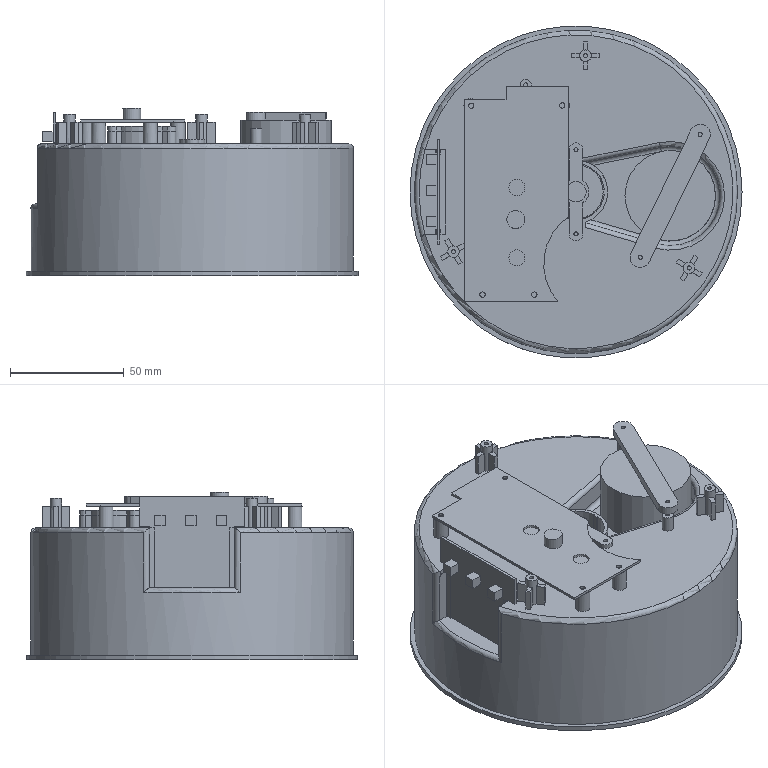Assembly | NX | mm | 9 component files | 9 solids | 350 faces | box 146 x 146 x 73.54 mm | volume 144346 mm3 | plane 205 | cylinder 113 | torus 18 | spline 7 | sphere 7 | commonest cylinder face diameters 4 x27 1.8 x17 2.35 x8 4.915 x6 24 x6 5 x5 23.94 x4 24.9 x4
Bill of materials:
unnamed part 1 | 1 |  | Thin flat plate with a T-shaped outline: a wider rectangular head band over a narrower rectangular body. The edge views show small rectangular blocks standing out from one face.
unnamed part 2 | 1 |  | Flat bar with rounded ends and a small through hole near each end. At the middle is a ring-shaped pad over a hollow cylindrical tube that sticks out from one side of the bar.
unnamed part 3 | 1 |  | Thin round disc with three rounded ears spaced about evenly around the edge. Each ear has a small through hole.
unnamed part 4 | 1 |  | Long, thin flat bar with rounded ends and a small through hole near each end.
unnamed part 5 | 1 |  | Wide, short cylindrical housing with a closed top and a narrow lip around the base. The top carries several upright features: small round posts, cross-shaped posts, a central boss with mounting lugs, and a hollow tube boss with a raised teardrop-shaped wall running from it.
unnamed part 6 | 1 |  | Solid cylinder with a short, narrower step collar on one end and a thin round shaft extending from the collar on the same axis.
unnamed part 7 | 1 |  | Plain solid cylinder, wider than it is tall.
unnamed part 8 | 1 |  | Thin flat plate, roughly rectangular, with a step-shaped notch along one short edge and a large curved (concave) cutout at one corner. It has two larger through holes, four small holes near the corners, and one short cylindrical boss standing on the top face.
unnamed part 9 | 1 |  | Plain solid disc whose diameter is several times its thickness.
Mates:
1. touch align | motor 1 face | inner_liner 1 face
2. distance | motor 1 face | inner_liner 1 face
3. distance | speaker 1 face | inner_liner 1 face
4. touch align | speaker_mount 1 face | speaker 1 face
5. touch align | atomizer_head 1 face | inner_liner 1 face
6. distance | pcb_large 1 face | inner_liner 1 face
7. center | pcb_small 1 face | pcb_small 1 face | inner_liner 1 face | inner_liner 1 face
8. touch align | pcb_small 1 face | inner_liner 1 face